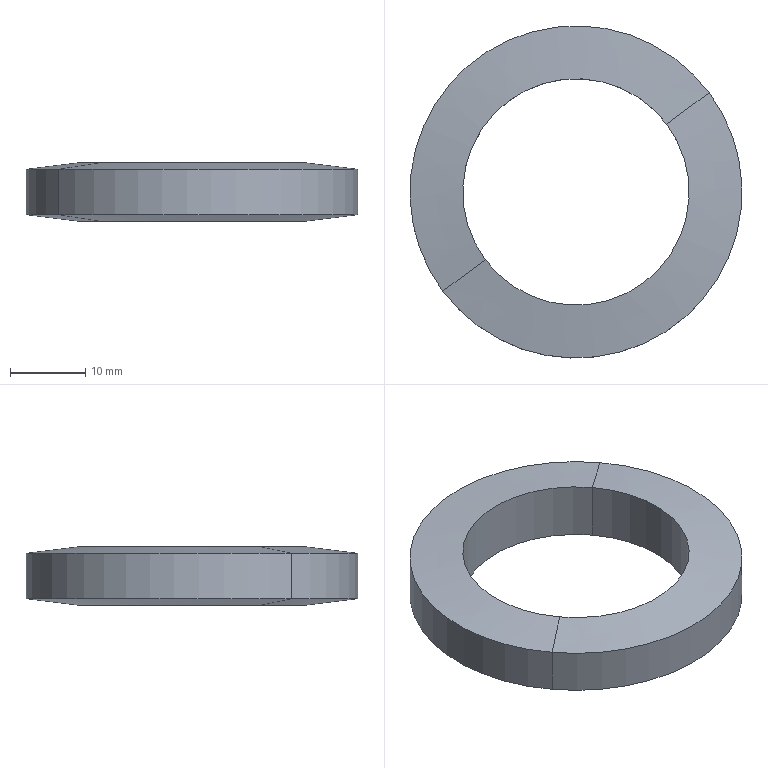Component | SolidWorks | 26-1 | 1 solid | 8 faces | box 44 x 44 x 7.72 mm | volume 5537 mm3 | cylinder 4 | cone 4 | commonest cylinder face diameters 30 x2 44 x2
build123d program:
from build123d import *


with BuildPart() as part:
    # Sketch1 → Revolve1 (revolve)
    with BuildSketch(Plane(origin=(0, 0, 0), x_dir=(1, 0, 0), z_dir=(0, 1, 0)), mode=Mode.PRIVATE) as revolve1_sk:
        Polygon((15, -3.859), (15, 3.859), (22, 3), (22, -3), align=None)
    revolve(revolve1_sk.sketch.rotate(Axis((0, 0, -15.97), (0, 0, 1)), 180), axis=Axis((0, 0, -15.97), (0, 0, 1)))


solid = part.part

# Placed as in the assembly
solid = solid.moved(Location((70, -47, -82.7), (0, 0, 0)))
STEP:
#1=COLOUR_RGB('',0.7922,0.8196,0.9333);
#2=FILL_AREA_STYLE_COLOUR('',#1);
#3=FILL_AREA_STYLE('',(#2));
#4=SURFACE_STYLE_FILL_AREA(#3);
#5=SURFACE_SIDE_STYLE('',(#4));
#6=SURFACE_STYLE_USAGE(.BOTH.,#5);
#7=PRESENTATION_STYLE_ASSIGNMENT((#6));
#8=CARTESIAN_POINT('',(3.229,-1.497,-3.408));
#9=VERTEX_POINT('',#8);
#10=CARTESIAN_POINT('',(2.283,-2.203,-3.408));
#11=VERTEX_POINT('',#10);
#12=CARTESIAN_POINT('',(2.756,-1.85,-3.408));
#13=DIRECTION('',(0.,0.,1.));
#14=DIRECTION('',(-0.8016,-0.5979,0.));
#15=AXIS2_PLACEMENT_3D('',#12,#13,#14);
#16=CIRCLE('',#15,0.5906);
#17=EDGE_CURVE('',#9,#11,#16,.T.);
#18=ORIENTED_EDGE('',*,*,#17,.F.);
#19=CARTESIAN_POINT('',(3.229,-1.497,-3.104));
#20=VERTEX_POINT('',#19);
#21=CARTESIAN_POINT('',(3.229,-1.497,-2.627));
#22=DIRECTION('',(0.,0.,1.));
#23=VECTOR('',#22,39.37);
#24=LINE('',#21,#23);
#25=EDGE_CURVE('',#9,#20,#24,.T.);
#26=ORIENTED_EDGE('',*,*,#25,.T.);
#27=CARTESIAN_POINT('',(2.283,-2.203,-3.104));
#28=VERTEX_POINT('',#27);
#29=CARTESIAN_POINT('',(2.756,-1.85,-3.104));
#30=DIRECTION('',(0.,0.,1.));
#31=DIRECTION('',(-0.8016,-0.5979,0.));
#32=AXIS2_PLACEMENT_3D('',#29,#30,#31);
#33=CIRCLE('',#32,0.5906);
#34=EDGE_CURVE('',#20,#28,#33,.T.);
#35=ORIENTED_EDGE('',*,*,#34,.T.);
#36=CARTESIAN_POINT('',(2.283,-2.203,-2.627));
#37=DIRECTION('',(0.,0.,1.));
#38=VECTOR('',#37,39.37);
#39=LINE('',#36,#38);
#40=EDGE_CURVE('',#11,#28,#39,.T.);
#41=ORIENTED_EDGE('',*,*,#40,.F.);
#42=EDGE_LOOP('',(#18,#26,#35,#41));
#43=FACE_OUTER_BOUND('',#42,.T.);
#44=CARTESIAN_POINT('',(2.756,-1.85,-2.627));
#45=DIRECTION('',(0.,0.,1.));
#46=DIRECTION('',(-0.8016,-0.5979,0.));
#47=AXIS2_PLACEMENT_3D('',#44,#45,#46);
#48=CYLINDRICAL_SURFACE('',#47,0.5906);
#49=ADVANCED_FACE('',(#43),#48,.F.);
#50=CARTESIAN_POINT('',(2.756,-1.85,-3.408));
#51=DIRECTION('',(0.,0.,1.));
#52=DIRECTION('',(-0.8016,-0.5979,0.));
#53=AXIS2_PLACEMENT_3D('',#50,#51,#52);
#54=CIRCLE('',#53,0.5906);
#55=EDGE_CURVE('',#11,#9,#54,.T.);
#56=ORIENTED_EDGE('',*,*,#55,.T.);
#57=CARTESIAN_POINT('',(3.45,-1.333,-3.374));
#58=VERTEX_POINT('',#57);
#59=CARTESIAN_POINT('',(3.229,-1.497,-3.408));
#60=DIRECTION('',(0.7956,0.5934,0.1219));
#61=VECTOR('',#60,39.37);
#62=LINE('',#59,#61);
#63=EDGE_CURVE('',#9,#58,#62,.T.);
#64=ORIENTED_EDGE('',*,*,#63,.T.);
#65=CARTESIAN_POINT('',(2.062,-2.368,-3.374));
#66=VERTEX_POINT('',#65);
#67=CARTESIAN_POINT('',(2.756,-1.85,-3.374));
#68=DIRECTION('',(0.,0.,1.));
#69=DIRECTION('',(-0.8016,-0.5979,0.));
#70=AXIS2_PLACEMENT_3D('',#67,#68,#69);
#71=CIRCLE('',#70,0.8661);
#72=EDGE_CURVE('',#66,#58,#71,.T.);
#73=ORIENTED_EDGE('',*,*,#72,.F.);
#74=CARTESIAN_POINT('',(2.283,-2.203,-3.408));
#75=DIRECTION('',(-0.7956,-0.5934,0.1219));
#76=VECTOR('',#75,39.37);
#77=LINE('',#74,#76);
#78=EDGE_CURVE('',#11,#66,#77,.T.);
#79=ORIENTED_EDGE('',*,*,#78,.F.);
#80=EDGE_LOOP('',(#56,#64,#73,#79));
#81=FACE_OUTER_BOUND('',#80,.T.);
#82=CARTESIAN_POINT('',(2.756,-1.85,-3.408));
#83=DIRECTION('',(0.,0.,1.));
#84=DIRECTION('',(-0.8016,-0.5979,0.));
#85=AXIS2_PLACEMENT_3D('',#82,#83,#84);
#86=CONICAL_SURFACE('',#85,0.5906,1.449);
#87=ADVANCED_FACE('',(#81),#86,.T.);
#88=ORIENTED_EDGE('',*,*,#72,.T.);
#89=CARTESIAN_POINT('',(3.45,-1.333,-3.138));
#90=VERTEX_POINT('',#89);
#91=CARTESIAN_POINT('',(3.45,-1.333,-2.627));
#92=DIRECTION('',(0.,0.,1.));
#93=VECTOR('',#92,39.37);
#94=LINE('',#91,#93);
#95=EDGE_CURVE('',#58,#90,#94,.T.);
#96=ORIENTED_EDGE('',*,*,#95,.T.);
#97=CARTESIAN_POINT('',(2.062,-2.368,-3.138));
#98=VERTEX_POINT('',#97);
#99=CARTESIAN_POINT('',(2.756,-1.85,-3.138));
#100=DIRECTION('',(0.,0.,1.));
#101=DIRECTION('',(-0.8016,-0.5979,0.));
#102=AXIS2_PLACEMENT_3D('',#99,#100,#101);
#103=CIRCLE('',#102,0.8661);
#104=EDGE_CURVE('',#98,#90,#103,.T.);
#105=ORIENTED_EDGE('',*,*,#104,.F.);
#106=CARTESIAN_POINT('',(2.062,-2.368,-2.627));
#107=DIRECTION('',(0.,0.,1.));
#108=VECTOR('',#107,39.37);
#109=LINE('',#106,#108);
#110=EDGE_CURVE('',#66,#98,#109,.T.);
#111=ORIENTED_EDGE('',*,*,#110,.F.);
#112=EDGE_LOOP('',(#88,#96,#105,#111));
#113=FACE_OUTER_BOUND('',#112,.T.);
#114=CARTESIAN_POINT('',(2.756,-1.85,-2.627));
#115=DIRECTION('',(0.,0.,1.));
#116=DIRECTION('',(-0.8016,-0.5979,0.));
#117=AXIS2_PLACEMENT_3D('',#114,#115,#116);
#118=CYLINDRICAL_SURFACE('',#117,0.8661);
#119=ADVANCED_FACE('',(#113),#118,.T.);
#120=CARTESIAN_POINT('',(2.756,-1.85,-3.104));
#121=DIRECTION('',(0.,0.,1.));
#122=DIRECTION('',(-0.8016,-0.5979,0.));
#123=AXIS2_PLACEMENT_3D('',#120,#121,#122);
#124=CIRCLE('',#123,0.5906);
#125=EDGE_CURVE('',#28,#20,#124,.T.);
#126=ORIENTED_EDGE('',*,*,#125,.F.);
#127=CARTESIAN_POINT('',(2.062,-2.368,-3.138));
#128=DIRECTION('',(-0.7956,-0.5934,-0.1219));
#129=VECTOR('',#128,39.37);
#130=LINE('',#127,#129);
#131=EDGE_CURVE('',#28,#98,#130,.T.);
#132=ORIENTED_EDGE('',*,*,#131,.T.);
#133=ORIENTED_EDGE('',*,*,#104,.T.);
#134=CARTESIAN_POINT('',(3.45,-1.333,-3.138));
#135=DIRECTION('',(0.7956,0.5934,-0.1219));
#136=VECTOR('',#135,39.37);
#137=LINE('',#134,#136);
#138=EDGE_CURVE('',#20,#90,#137,.T.);
#139=ORIENTED_EDGE('',*,*,#138,.F.);
#140=EDGE_LOOP('',(#126,#132,#133,#139));
#141=FACE_OUTER_BOUND('',#140,.T.);
#142=CARTESIAN_POINT('',(2.756,-1.85,-3.138));
#143=DIRECTION('',(-0.,-0.,-1.));
#144=DIRECTION('',(0.8016,0.5979,-0.));
#145=AXIS2_PLACEMENT_3D('',#142,#143,#144);
#146=CONICAL_SURFACE('',#145,0.8661,1.449);
#147=ADVANCED_FACE('',(#141),#146,.T.);
#148=ORIENTED_EDGE('',*,*,#131,.F.);
#149=ORIENTED_EDGE('',*,*,#34,.F.);
#150=ORIENTED_EDGE('',*,*,#138,.T.);
#151=CARTESIAN_POINT('',(2.756,-1.85,-3.138));
#152=DIRECTION('',(0.,0.,1.));
#153=DIRECTION('',(-0.8016,-0.5979,0.));
#154=AXIS2_PLACEMENT_3D('',#151,#152,#153);
#155=CIRCLE('',#154,0.8661);
#156=EDGE_CURVE('',#90,#98,#155,.T.);
#157=ORIENTED_EDGE('',*,*,#156,.T.);
#158=EDGE_LOOP('',(#148,#149,#150,#157));
#159=FACE_OUTER_BOUND('',#158,.T.);
#160=CARTESIAN_POINT('',(2.756,-1.85,-3.138));
#161=DIRECTION('',(-0.,-0.,-1.));
#162=DIRECTION('',(0.8016,0.5979,-0.));
#163=AXIS2_PLACEMENT_3D('',#160,#161,#162);
#164=CONICAL_SURFACE('',#163,0.8661,1.449);
#165=ADVANCED_FACE('',(#159),#164,.T.);
#166=ORIENTED_EDGE('',*,*,#95,.F.);
#167=CARTESIAN_POINT('',(2.756,-1.85,-3.374));
#168=DIRECTION('',(0.,0.,1.));
#169=DIRECTION('',(-0.8016,-0.5979,0.));
#170=AXIS2_PLACEMENT_3D('',#167,#168,#169);
#171=CIRCLE('',#170,0.8661);
#172=EDGE_CURVE('',#58,#66,#171,.T.);
#173=ORIENTED_EDGE('',*,*,#172,.T.);
#174=ORIENTED_EDGE('',*,*,#110,.T.);
#175=ORIENTED_EDGE('',*,*,#156,.F.);
#176=EDGE_LOOP('',(#166,#173,#174,#175));
#177=FACE_OUTER_BOUND('',#176,.T.);
#178=CARTESIAN_POINT('',(2.756,-1.85,-2.627));
#179=DIRECTION('',(0.,0.,1.));
#180=DIRECTION('',(-0.8016,-0.5979,0.));
#181=AXIS2_PLACEMENT_3D('',#178,#179,#180);
#182=CYLINDRICAL_SURFACE('',#181,0.8661);
#183=ADVANCED_FACE('',(#177),#182,.T.);
#184=ORIENTED_EDGE('',*,*,#63,.F.);
#185=ORIENTED_EDGE('',*,*,#17,.T.);
#186=ORIENTED_EDGE('',*,*,#78,.T.);
#187=ORIENTED_EDGE('',*,*,#172,.F.);
#188=EDGE_LOOP('',(#184,#185,#186,#187));
#189=FACE_OUTER_BOUND('',#188,.T.);
#190=CARTESIAN_POINT('',(2.756,-1.85,-3.408));
#191=DIRECTION('',(0.,0.,1.));
#192=DIRECTION('',(-0.8016,-0.5979,0.));
#193=AXIS2_PLACEMENT_3D('',#190,#191,#192);
#194=CONICAL_SURFACE('',#193,0.5906,1.449);
#195=ADVANCED_FACE('',(#189),#194,.T.);
#196=ORIENTED_EDGE('',*,*,#25,.F.);
#197=ORIENTED_EDGE('',*,*,#55,.F.);
#198=ORIENTED_EDGE('',*,*,#40,.T.);
#199=ORIENTED_EDGE('',*,*,#125,.T.);
#200=EDGE_LOOP('',(#196,#197,#198,#199));
#201=FACE_OUTER_BOUND('',#200,.T.);
#202=CARTESIAN_POINT('',(2.756,-1.85,-2.627));
#203=DIRECTION('',(0.,0.,1.));
#204=DIRECTION('',(-0.8016,-0.5979,0.));
#205=AXIS2_PLACEMENT_3D('',#202,#203,#204);
#206=CYLINDRICAL_SURFACE('',#205,0.5906);
#207=ADVANCED_FACE('',(#201),#206,.F.);
#208=CLOSED_SHELL('',(#49,#87,#119,#147,#165,#183,#195,#207));
#209=MANIFOLD_SOLID_BREP('',#208);
#210=STYLED_ITEM('',(#7),#209);
#211=(LENGTH_UNIT()NAMED_UNIT(*)SI_UNIT($,.METRE.));
#212=LENGTH_MEASURE_WITH_UNIT(LENGTH_MEASURE(0.0254),#211);
#213=DIMENSIONAL_EXPONENTS(1.,0.,0.,0.,0.,0.,0.);
#214=(CONVERSION_BASED_UNIT('',#212)LENGTH_UNIT()NAMED_UNIT(#213));
#215=UNCERTAINTY_MEASURE_WITH_UNIT(LENGTH_MEASURE(0.00001),#214,'','');
#216=(NAMED_UNIT(*)PLANE_ANGLE_UNIT()SI_UNIT($,.RADIAN.));
#217=(NAMED_UNIT(*)SI_UNIT($,.STERADIAN.)SOLID_ANGLE_UNIT());
#218=(GEOMETRIC_REPRESENTATION_CONTEXT(3)GLOBAL_UNCERTAINTY_ASSIGNED_CONTEXT((#215))GLOBAL_UNIT_ASSIGNED_CONTEXT((#214,#216,#217))REPRESENTATION_CONTEXT('',''));
#219=MECHANICAL_DESIGN_GEOMETRIC_PRESENTATION_REPRESENTATION('',(#210),#218);
#220=PRESENTATION_LAYER_ASSIGNMENT('','',(#210));
#221=CARTESIAN_POINT('',(0.,0.,0.));
#222=DIRECTION('',(0.,0.,1.));
#223=DIRECTION('',(1.,0.,0.));
#224=AXIS2_PLACEMENT_3D('',#221,#222,#223);
#225=(LENGTH_UNIT()NAMED_UNIT(*)SI_UNIT($,.METRE.));
#226=LENGTH_MEASURE_WITH_UNIT(LENGTH_MEASURE(0.0254),#225);
#227=DIMENSIONAL_EXPONENTS(1.,0.,0.,0.,0.,0.,0.);
#228=(CONVERSION_BASED_UNIT('',#226)LENGTH_UNIT()NAMED_UNIT(#227));
#229=UNCERTAINTY_MEASURE_WITH_UNIT(LENGTH_MEASURE(0.00001),#228,'','');
#230=(NAMED_UNIT(*)PLANE_ANGLE_UNIT()SI_UNIT($,.RADIAN.));
#231=(NAMED_UNIT(*)SI_UNIT($,.STERADIAN.)SOLID_ANGLE_UNIT());
#232=(GEOMETRIC_REPRESENTATION_CONTEXT(3)GLOBAL_UNCERTAINTY_ASSIGNED_CONTEXT((#229))GLOBAL_UNIT_ASSIGNED_CONTEXT((#228,#230,#231))REPRESENTATION_CONTEXT('',''));
#233=ADVANCED_BREP_SHAPE_REPRESENTATION('',(#209,#224),#232);